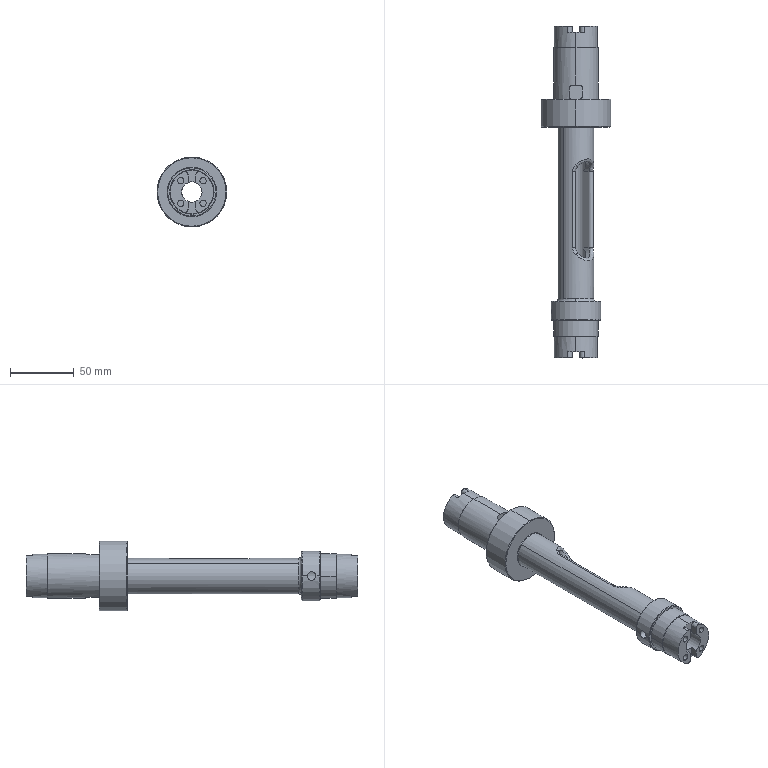CAM job | Mastercam | mm | 6 operations | part box 55 x 261 x 55
1. 3D High Speed (Area roughing) | 10 - 10 平铣刀
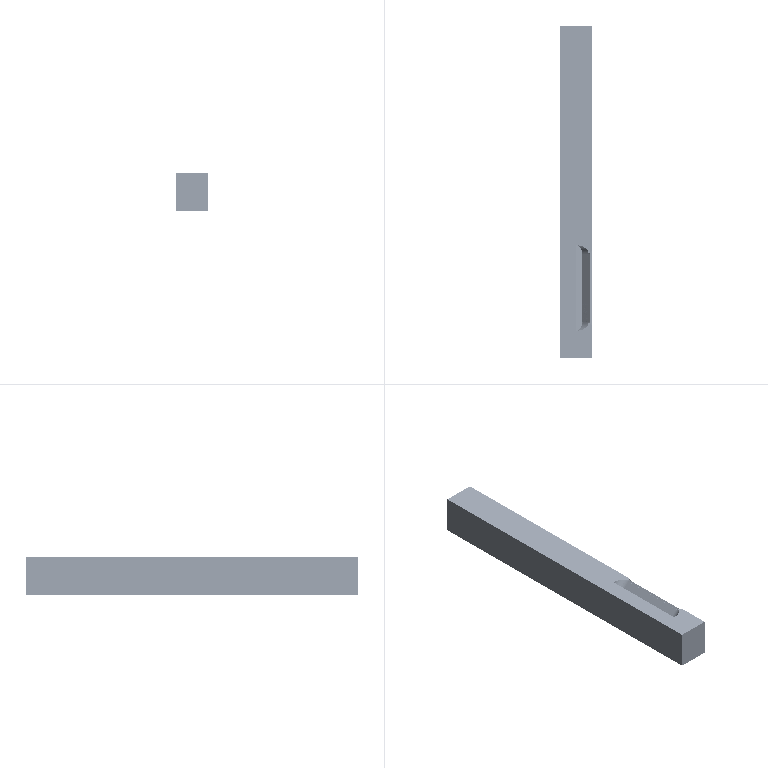2. Unified Morph | 5 - 6 球刀/圆鼻铣刀
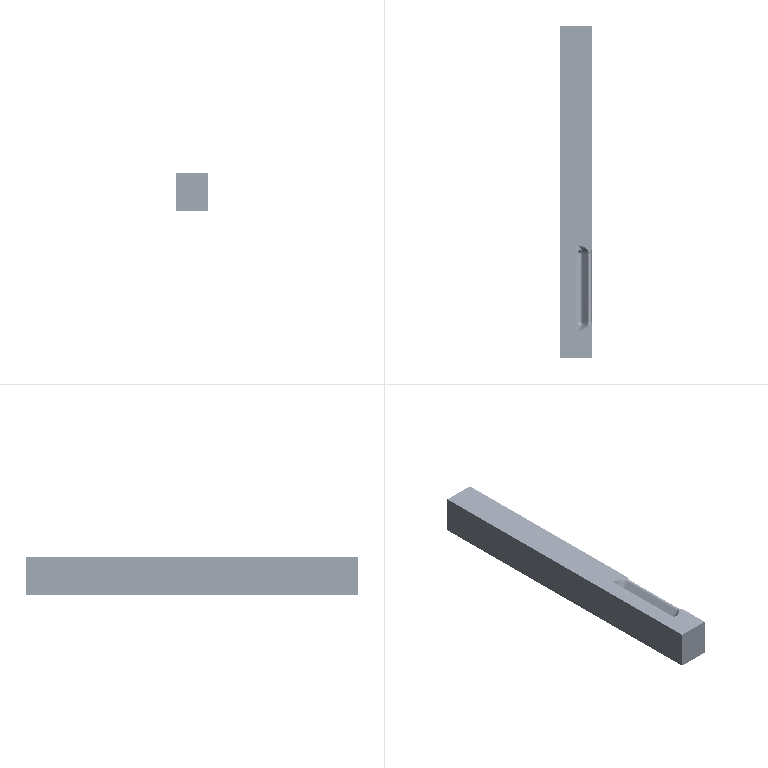3. Drill/Counterbore | 7 - 4 倒角刀
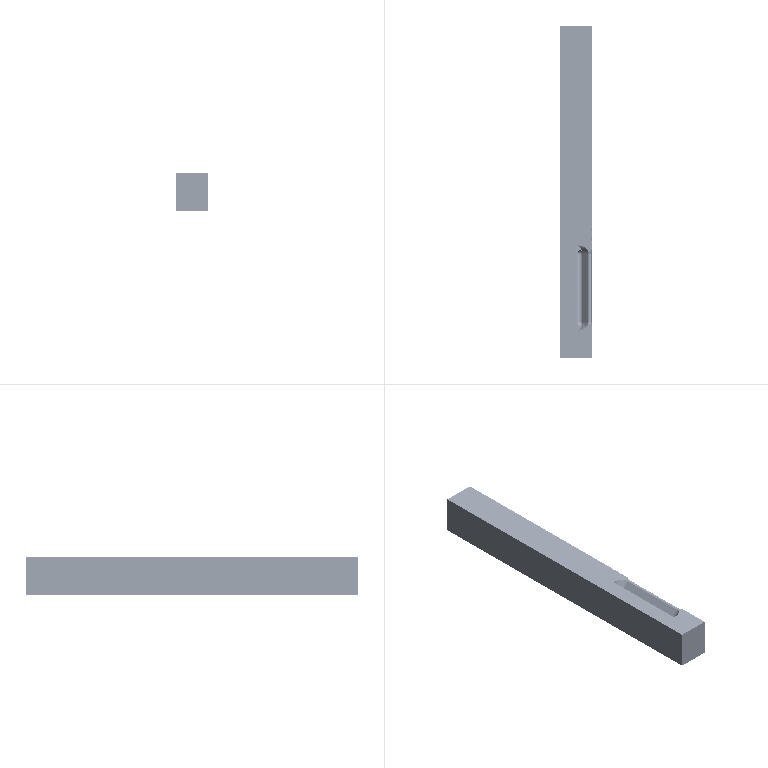4. Peck Drill | 1 - 2.5 钻头
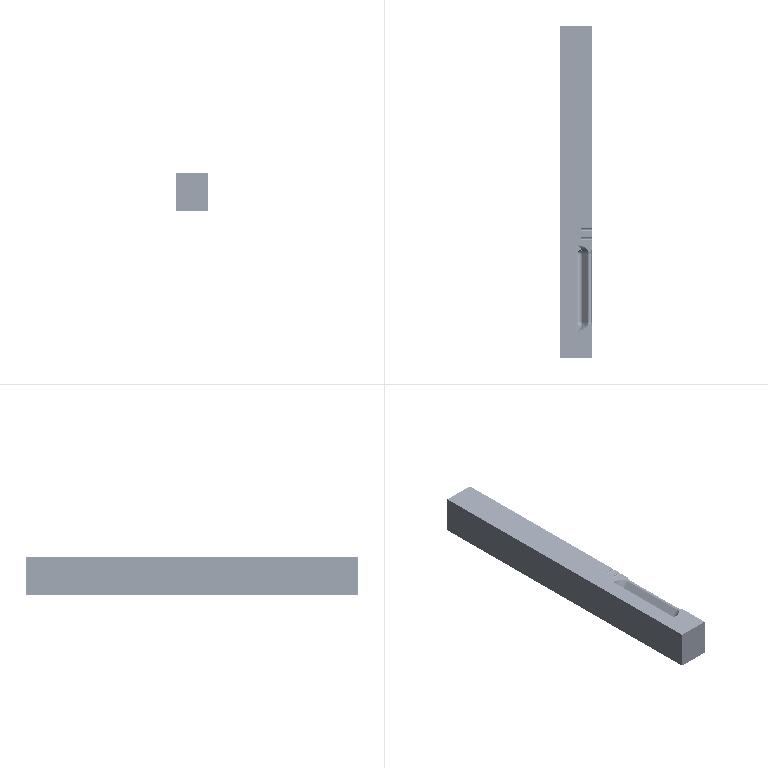5. Drill/Counterbore | 7 - 4 倒角刀
6. Peck Drill | 17 - 7 钻头